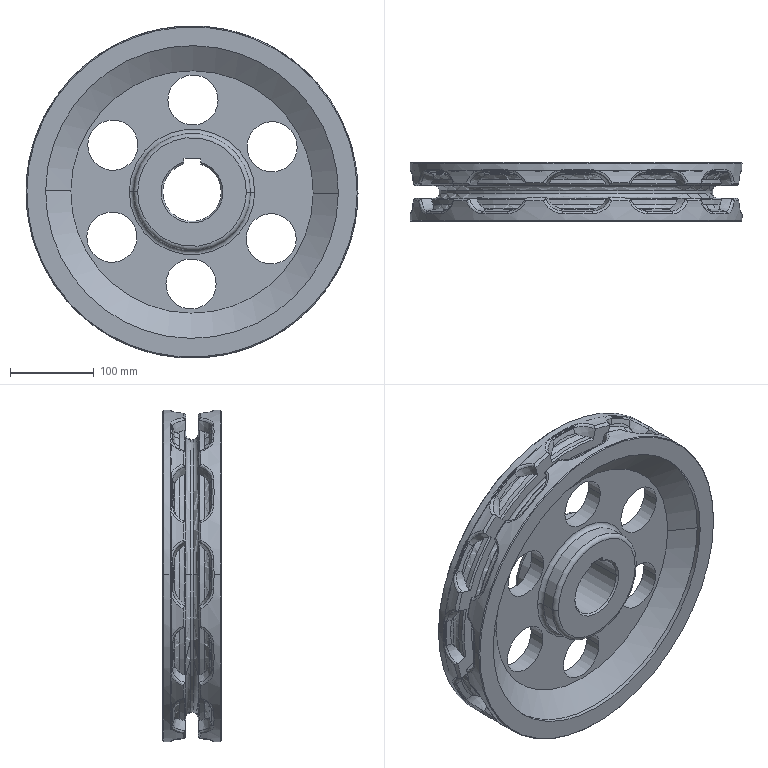Component | SolidWorks | LowerTensioningDeviceAssembly-1_DriveSprocket-Driven2-1 | 1 solid | 344 faces | volume 3712896 mm3 | cone 144 | spline 72 | cylinder 55 | torus 38 | plane 35 | commonest cylinder face diameters 367 x26 60 x12 140 x4 350 x4 397 x4 70 x3 327 x2